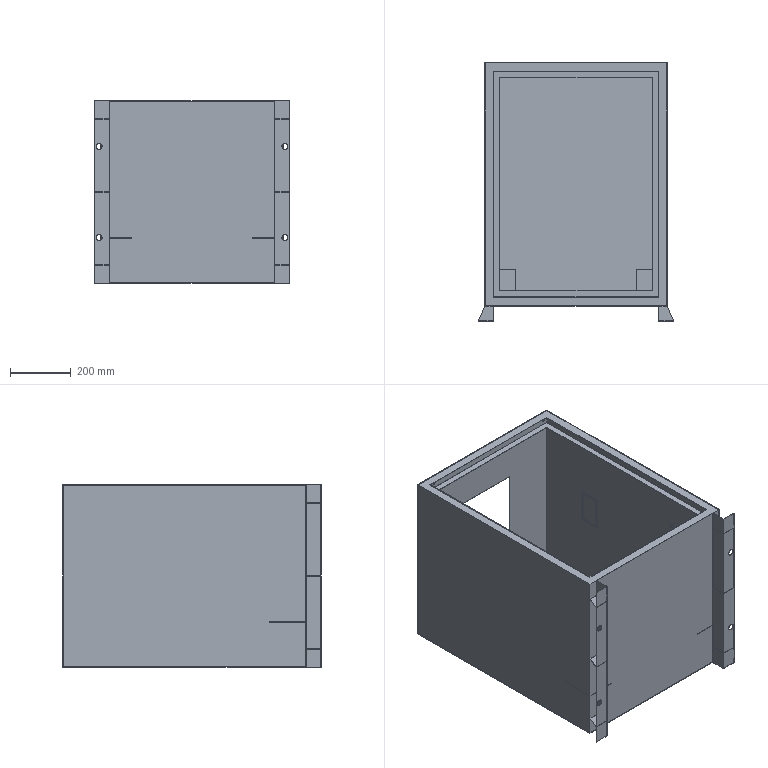Component | SolidWorks | Box-1 | 1 solid | 140 faces | box 640 x 850 x 600 mm | volume 3637443 mm3 | plane 124 | cylinder 16 | commonest cylinder face diameters 20 x8 10 x4 5 x4
build123d program:
from build123d import *

# Parameters (mm, degrees)
SKETCH1_2_W           = 600
SKETCH1_2_H           = 600
BOSS_EXTRUDE1_2_DEPTH = 800
SHELL1_T              = -1.5
SKETCH3_W             = 600
SKETCH3_H             = 800
SKETCH3_W_2           = 540
SKETCH3_H_2           = 740
BOSS_EXTRUDE2_2_DEPTH = 1.5
SKETCH4_W             = 20
SKETCH4_H             = 740
BOSS_EXTRUDE3_DEPTH   = 1.5
SKETCH5_2_W           = 540
SKETCH5_2_H           = 18.5
BOSS_EXTRUDE6_DEPTH   = 1.5
SKETCH6_2_W           = 543
SKETCH6_2_H           = 743
SKETCH6_2_W_2         = 500
SKETCH6_2_H_2         = 700
BOSS_EXTRUDE7_DEPTH   = 1.5
SKETCH7_W             = 600
SKETCH7_H             = 50
BOSS_EXTRUDE8_DEPTH   = 1.5
SKETCH9_W             = 50
SKETCH9_H             = 600
BOSS_EXTRUDE10_DEPTH  = 1.5
BOSS_EXTRUDE11_DEPTH  = 0.75
LPATTERN1_COUNT       = 2
LPATTERN1_PITCH       = 240
LPATTERN1_COL_COUNT   = 2
LPATTERN1_COL_PITCH   = 240
SKETCH11_R            = 10
CUT_EXTRUDE1_2_DEPTH  = 1.5
MIRROR3_COPY_1_DEPTH  = 0.75
MIRROR3_COPY_2_DEPTH  = 0.75
SKETCH23_W            = 1.5
SKETCH23_H            = 120
BOSS_EXTRUDE15_DEPTH  = 100
SKETCH24_W            = 5
SKETCH24_H            = 5
CUT_EXTRUDE8_DEPTH    = 10
SKETCH12_W            = 247
SKETCH12_H            = 235
CUT_EXTRUDE9_DEPTH    = 10
SKETCH25_W            = 254
SKETCH25_H            = 242
SKETCH25_W_2          = 251
SKETCH25_H_2          = 239
BOSS_EXTRUDE16_DEPTH  = 50
SKETCH26_W            = 133
SKETCH26_H            = 12
CUT_EXTRUDE10_DEPTH   = 10
SKETCH27_W            = 251
SKETCH27_H            = 239
CUT_EXTRUDE11_DEPTH   = 10
SKETCH1_W             = 254
SKETCH1_H             = 78.653
CUT_EXTRUDE1_DEPTH    = 1002.07
SKETCH5_R             = 5
SKETCH5_R_2           = 2.5
BOSS_EXTRUDE1_DEPTH   = 5
SKETCH6_W             = 110
SKETCH6_H             = 70
SKETCH6_W_2           = 100
SKETCH6_H_2           = 60
BOSS_EXTRUDE2_DEPTH   = 3
CHAMFER1_SIZE         = 1


with BuildPart() as part:
    # Sketch1_2 → Boss-Extrude1_2 (new body)
    with BuildSketch(Plane(origin=(0, 0, 0), x_dir=(1, 0, 0), z_dir=(0, 1, 0))):
        Rectangle(SKETCH1_2_W, SKETCH1_2_H)
    extrude(amount=BOSS_EXTRUDE1_2_DEPTH)

    # Shell1
    shell1_openings = [part.faces().sort_by_distance(p)[0] for p in [
        (0, 400, 300),
    ]]
    offset(amount=SHELL1_T, openings=shell1_openings, kind=Kind.INTERSECTION)

    # Sketch3 → Boss-Extrude2_2 (add)
    with BuildSketch(Plane.XY.offset(300)):
        with Locations((0, 400)):
            Rectangle(SKETCH3_W, SKETCH3_H)
        with Locations((0, 400)):
            Rectangle(SKETCH3_W_2, SKETCH3_H_2, mode=Mode.SUBTRACT)
    extrude(amount=-BOSS_EXTRUDE2_2_DEPTH)

    # Sketch4 → Boss-Extrude3 (add)
    with BuildSketch(Plane(origin=(-270, 0, 0), x_dir=(0, 0, -1), z_dir=(1, 0, 0))):
        with Locations((-290, 400)):
            Rectangle(SKETCH4_W, SKETCH4_H)
    boss_extrude3 = extrude(amount=-BOSS_EXTRUDE3_DEPTH)

    # Sketch5_2 → Boss-Extrude6 (add)
    with BuildSketch(Plane(origin=(0, 30, 0), x_dir=(1, 0, 0), z_dir=(0, 1, 0))):
        Polygon((-271.5, -300), (-270, -300), (-270, -298.5), (-270, -280), (-271.5, -280), align=None)
        Polygon((270, -298.5), (270, -300), (271.5, -300), (271.5, -280), (270, -280), align=None)
        with Locations((0, -289.25)):
            Rectangle(SKETCH5_2_W, SKETCH5_2_H)
    boss_extrude6 = extrude(amount=-BOSS_EXTRUDE6_DEPTH)

    # Mirror1: Boss-Extrude6 across plane
    add(boss_extrude6.mirror(Plane.ZX.offset(400)))

    # Mirror2: Boss-Extrude3 across plane
    add(boss_extrude3.mirror(Plane(origin=(0, 0, 0), x_dir=(0, 0, 1), z_dir=(1, 0, 0))))

    # Sketch6_2 → Boss-Extrude7 (add)
    with BuildSketch(Plane(origin=(0, 0, 280), x_dir=(-1, 0, 0), z_dir=(0, 0, -1))):
        with Locations((0, 400)):
            Rectangle(SKETCH6_2_W, SKETCH6_2_H)
        with Locations((0, 400)):
            Rectangle(SKETCH6_2_W_2, SKETCH6_2_H_2, mode=Mode.SUBTRACT)
    extrude(amount=BOSS_EXTRUDE7_DEPTH)

    # Sketch7 → Boss-Extrude8 (add)
    with BuildSketch(Plane.ZY.offset(-270)):
        with Locations((0, -25)):
            Rectangle(SKETCH7_W, SKETCH7_H)
    boss_extrude8 = extrude(amount=-BOSS_EXTRUDE8_DEPTH)

    # Sketch9 → Boss-Extrude10 (add)
    with BuildSketch(Plane.XZ.offset(50)):
        with Locations((295, 0)):
            Rectangle(SKETCH9_W, SKETCH9_H)
    boss_extrude10 = extrude(amount=-BOSS_EXTRUDE10_DEPTH)

    # Sketch10 → Boss-Extrude11 (add, symmetric)
    with BuildSketch(Plane.XY):
        Polygon((271.5, -48.5), (271.5, 0), (300, 0), (320, -48.5), align=None)
    boss_extrude11 = extrude(amount=BOSS_EXTRUDE11_DEPTH, both=True)

    # LPattern1: Boss-Extrude11 ×2
    with Locations(*[(0, 0, i * LPATTERN1_PITCH) for i in range(1, LPATTERN1_COUNT)]):
        add(boss_extrude11)

    # LPattern1 col: Boss-Extrude11 ×2
    with Locations(*[(0, 0, -i * LPATTERN1_COL_PITCH) for i in range(1, LPATTERN1_COL_COUNT)]):
        add(boss_extrude11)

    # Sketch11 → Cut-Extrude1_2 (cut, symmetric)
    with BuildSketch(Plane(origin=(0, -48.5, 0), x_dir=(1, 0, 0), z_dir=(0, 1, 0))):
        with Locations(Location((305, -150, 0), (0, 0, 270))):
            Circle(SKETCH11_R)
        with Locations(Location((305, 150, 0), (0, 0, 90))):
            Circle(SKETCH11_R)
    cut_extrude1_2 = extrude(amount=CUT_EXTRUDE1_2_DEPTH, both=True, mode=Mode.SUBTRACT)

    # Mirror3: Boss-Extrude8, Boss-Extrude10, Boss-Extrude11, Cut-Extrude1_2 across plane
    add(boss_extrude8.mirror(Plane(origin=(0, 0, 0), x_dir=(0, 0, 1), z_dir=(1, 0, 0))))
    add(boss_extrude10.mirror(Plane(origin=(0, 0, 0), x_dir=(0, 0, 1), z_dir=(1, 0, 0))))
    add(boss_extrude11.mirror(Plane(origin=(0, 0, 0), x_dir=(0, 0, 1), z_dir=(1, 0, 0))))
    add(cut_extrude1_2.mirror(Plane(origin=(0, 0, 0), x_dir=(0, 0, 1), z_dir=(1, 0, 0))), mode=Mode.SUBTRACT)

    # Mirror3 copy 1 sketch → Mirror3 copy 1 (add, symmetric)
    with BuildSketch(Plane(origin=(0, 0, 240), x_dir=(-1, 0, 0), z_dir=(0, 0, 1))):
        Polygon((271.5, 48.5), (271.5, 0), (300, 0), (320, 48.5), align=None)
    extrude(amount=MIRROR3_COPY_1_DEPTH, both=True)

    # Mirror3 copy 2 sketch → Mirror3 copy 2 (add, symmetric)
    with BuildSketch(Plane(origin=(0, 0, -240), x_dir=(-1, 0, 0), z_dir=(0, 0, 1))):
        Polygon((271.5, 48.5), (271.5, 0), (300, 0), (320, 48.5), align=None)
    extrude(amount=MIRROR3_COPY_2_DEPTH, both=True)

    # Sketch23 → Boss-Extrude15 (add)
    with BuildSketch(Plane.ZY.offset(-298.5)):
        with Locations((-150.75, 61.5)):
            Rectangle(SKETCH23_W, SKETCH23_H)
    boss_extrude15 = extrude(amount=BOSS_EXTRUDE15_DEPTH)

    # Sketch24 → Cut-Extrude8 (cut)
    with BuildSketch(Plane(origin=(0, 30, 0), x_dir=(1, 0, 0), z_dir=(0, 1, 0))):
        with Locations((-255, -295)):
            Rectangle(SKETCH24_W, SKETCH24_H)
        with Locations((255, -295)):
            Rectangle(SKETCH24_W, SKETCH24_H)
    cut_extrude8 = extrude(amount=-CUT_EXTRUDE8_DEPTH, mode=Mode.SUBTRACT)

    # Mirror4: Cut-Extrude8 across plane
    add(cut_extrude8.mirror(Plane(origin=(0, 400, 0), x_dir=(0, 0, 1), z_dir=(0, -1, 0))), mode=Mode.SUBTRACT)

    # Sketch12 → Cut-Extrude9 (cut)
    with BuildSketch(Plane(origin=(0, 800, 0), x_dir=(1, 0, 0), z_dir=(0, 1, 0))):
        Rectangle(SKETCH12_W, SKETCH12_H)
    extrude(amount=-CUT_EXTRUDE9_DEPTH, mode=Mode.SUBTRACT)

    # Mirror5: Boss-Extrude15 across plane
    add(boss_extrude15.mirror(Plane(origin=(0, 0, 0), x_dir=(0, 0, 1), z_dir=(1, 0, 0))))

    # Sketch27 → Cut-Extrude11 (cut)
    with BuildSketch(Plane(origin=(0, 800, 0), x_dir=(1, 0, 0), z_dir=(0, 1, 0))):
        Rectangle(SKETCH27_W, SKETCH27_H)
    extrude(amount=-CUT_EXTRUDE11_DEPTH, mode=Mode.SUBTRACT)

    # Sketch5 → Boss-Extrude1 (add)
    # profile 1 of 2: a face of its own
    with BuildSketch(Plane.ZY.offset(-298.5)):
        with Locations((-145, 220)):
            Circle(SKETCH5_R)
        with Locations((-145, 220)):
            Circle(SKETCH5_R_2, mode=Mode.SUBTRACT)
    # profile 2 of 2: a face of its own
    with BuildSketch(Plane.ZY.offset(-298.5)):
        with Locations((125, 220)):
            Circle(SKETCH5_R)
        with Locations((125, 220)):
            Circle(SKETCH5_R_2, mode=Mode.SUBTRACT)
    extrude(amount=BOSS_EXTRUDE1_DEPTH)

    # Sketch6 → Boss-Extrude2 (add)
    with BuildSketch(Plane.ZY.offset(-298.5)):
        with Locations((0, 600)):
            Rectangle(SKETCH6_W, SKETCH6_H)
        with Locations((0, 600)):
            Rectangle(SKETCH6_W_2, SKETCH6_H_2, mode=Mode.SUBTRACT)
    extrude(amount=BOSS_EXTRUDE2_DEPTH)

    # Chamfer1
    chamfer1_edges = [part.edges().sort_by_distance(p)[0] for p in [
        (295.5, 600, 55),
        (295.5, 635, 0),
        (295.5, 600, -55),
        (295.5, 565, 0),
        (295.5, 630, 0),
        (295.5, 600, -50),
        (295.5, 570, 0),
        (295.5, 600, 50),
    ]]
    chamfer(chamfer1_edges, length=CHAMFER1_SIZE)


with BuildPart() as body_2:
    # Sketch25 → Boss-Extrude16 (new body)
    with BuildSketch(Plane(origin=(0, 800, 0), x_dir=(1, 0, 0), z_dir=(0, 1, 0))):
        Rectangle(SKETCH25_W, SKETCH25_H)
        Rectangle(SKETCH25_W_2, SKETCH25_H_2, mode=Mode.SUBTRACT)
    extrude(amount=BOSS_EXTRUDE16_DEPTH)

    # Sketch26 → Cut-Extrude10 (cut)
    with BuildSketch(Plane.XY.offset(121)):
        with Locations((0, 844)):
            Rectangle(SKETCH26_W, SKETCH26_H)
    extrude(amount=-CUT_EXTRUDE10_DEPTH, mode=Mode.SUBTRACT)

    # Sketch1 → Cut-Extrude1 (cut, through all)
    with BuildSketch(Plane.XY.offset(121)):
        with Locations((0, 839.326)):
            Rectangle(SKETCH1_W, SKETCH1_H)
    extrude(amount=-CUT_EXTRUDE1_DEPTH, mode=Mode.SUBTRACT)


solid = part.part